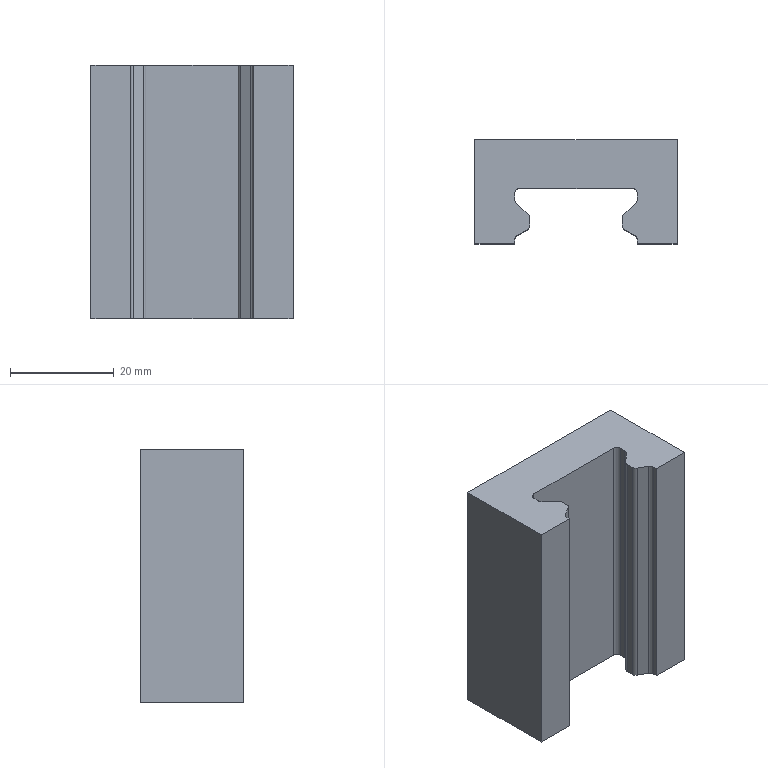Component | SolidWorks | MirrorSlider-2 | 1 solid | 28 faces | box 38.92 x 20 x 48.81 mm | volume 27036 mm3 | plane 18 | cylinder 10 | commonest cylinder face diameters 2 x10
STEP:
#1=COLOUR_RGB('',0.7922,0.8196,0.9333);
#2=FILL_AREA_STYLE_COLOUR('',#1);
#3=FILL_AREA_STYLE('',(#2));
#4=SURFACE_STYLE_FILL_AREA(#3);
#5=SURFACE_SIDE_STYLE('',(#4));
#6=SURFACE_STYLE_USAGE(.BOTH.,#5);
#7=PRESENTATION_STYLE_ASSIGNMENT((#6));
#8=CARTESIAN_POINT('',(-1.467,-8.441,-7.67));
#9=VERTEX_POINT('',#8);
#10=CARTESIAN_POINT('',(-1.467,-8.471,-7.67));
#11=VERTEX_POINT('',#10);
#12=CARTESIAN_POINT('',(-1.467,-7.683,-7.67));
#13=DIRECTION('',(0.,-1.,0.));
#14=VECTOR('',#13,39.37);
#15=LINE('',#12,#14);
#16=EDGE_CURVE('',#9,#11,#15,.T.);
#17=ORIENTED_EDGE('',*,*,#16,.F.);
#18=CARTESIAN_POINT('',(-1.486,-8.407,-7.67));
#19=VERTEX_POINT('',#18);
#20=CARTESIAN_POINT('',(-1.506,-8.441,-7.67));
#21=DIRECTION('',(0.,0.,1.));
#22=DIRECTION('',(0.,1.,0.));
#23=AXIS2_PLACEMENT_3D('',#20,#21,#22);
#24=CIRCLE('',#23,0.03937);
#25=EDGE_CURVE('',#9,#19,#24,.T.);
#26=ORIENTED_EDGE('',*,*,#25,.T.);
#27=CARTESIAN_POINT('',(-1.562,-8.363,-7.67));
#28=VERTEX_POINT('',#27);
#29=CARTESIAN_POINT('',(-0.6816,-8.869,-7.67));
#30=DIRECTION('',(0.8671,-0.4982,0.));
#31=VECTOR('',#30,39.37);
#32=LINE('',#29,#31);
#33=EDGE_CURVE('',#28,#19,#32,.T.);
#34=ORIENTED_EDGE('',*,*,#33,.F.);
#35=CARTESIAN_POINT('',(-1.582,-8.329,-7.67));
#36=VERTEX_POINT('',#35);
#37=CARTESIAN_POINT('',(-1.543,-8.329,-7.67));
#38=DIRECTION('',(0.,0.,1.));
#39=DIRECTION('',(0.,1.,0.));
#40=AXIS2_PLACEMENT_3D('',#37,#38,#39);
#41=CIRCLE('',#40,0.03937);
#42=EDGE_CURVE('',#36,#28,#41,.T.);
#43=ORIENTED_EDGE('',*,*,#42,.F.);
#44=CARTESIAN_POINT('',(-1.582,-8.278,-7.67));
#45=VERTEX_POINT('',#44);
#46=CARTESIAN_POINT('',(-1.582,-7.683,-7.67));
#47=DIRECTION('',(0.,-1.,0.));
#48=VECTOR('',#47,39.37);
#49=LINE('',#46,#48);
#50=EDGE_CURVE('',#45,#36,#49,.T.);
#51=ORIENTED_EDGE('',*,*,#50,.F.);
#52=CARTESIAN_POINT('',(-1.57,-8.249,-7.67));
#53=VERTEX_POINT('',#52);
#54=CARTESIAN_POINT('',(-1.543,-8.278,-7.67));
#55=DIRECTION('',(0.,0.,-1.));
#56=DIRECTION('',(0.,1.,0.));
#57=AXIS2_PLACEMENT_3D('',#54,#55,#56);
#58=CIRCLE('',#57,0.03937);
#59=EDGE_CURVE('',#45,#53,#58,.T.);
#60=ORIENTED_EDGE('',*,*,#59,.T.);
#61=CARTESIAN_POINT('',(-1.479,-8.164,-7.67));
#62=VERTEX_POINT('',#61);
#63=CARTESIAN_POINT('',(-0.4484,-7.203,-7.67));
#64=DIRECTION('',(-0.7311,-0.6823,0.));
#65=VECTOR('',#64,39.37);
#66=LINE('',#63,#65);
#67=EDGE_CURVE('',#62,#53,#66,.T.);
#68=ORIENTED_EDGE('',*,*,#67,.F.);
#69=CARTESIAN_POINT('',(-1.467,-8.136,-7.67));
#70=VERTEX_POINT('',#69);
#71=CARTESIAN_POINT('',(-1.506,-8.136,-7.67));
#72=DIRECTION('',(0.,0.,1.));
#73=DIRECTION('',(0.,1.,0.));
#74=AXIS2_PLACEMENT_3D('',#71,#72,#73);
#75=CIRCLE('',#74,0.03937);
#76=EDGE_CURVE('',#62,#70,#75,.T.);
#77=ORIENTED_EDGE('',*,*,#76,.T.);
#78=CARTESIAN_POINT('',(-1.467,-8.09,-7.67));
#79=VERTEX_POINT('',#78);
#80=CARTESIAN_POINT('',(-1.467,-7.683,-7.67));
#81=DIRECTION('',(0.,-1.,0.));
#82=VECTOR('',#81,39.37);
#83=LINE('',#80,#82);
#84=EDGE_CURVE('',#79,#70,#83,.T.);
#85=ORIENTED_EDGE('',*,*,#84,.F.);
#86=CARTESIAN_POINT('',(-1.506,-8.051,-7.67));
#87=VERTEX_POINT('',#86);
#88=CARTESIAN_POINT('',(-1.506,-8.09,-7.67));
#89=DIRECTION('',(0.,0.,-1.));
#90=DIRECTION('',(0.,1.,0.));
#91=AXIS2_PLACEMENT_3D('',#88,#89,#90);
#92=CIRCLE('',#91,0.03937);
#93=EDGE_CURVE('',#87,#79,#92,.T.);
#94=ORIENTED_EDGE('',*,*,#93,.F.);
#95=CARTESIAN_POINT('',(-2.356,-8.051,-7.67));
#96=VERTEX_POINT('',#95);
#97=CARTESIAN_POINT('',(-0.,-8.051,-7.67));
#98=DIRECTION('',(-1.,0.,0.));
#99=VECTOR('',#98,39.37);
#100=LINE('',#97,#99);
#101=EDGE_CURVE('',#87,#96,#100,.T.);
#102=ORIENTED_EDGE('',*,*,#101,.T.);
#103=CARTESIAN_POINT('',(-2.396,-8.09,-7.67));
#104=VERTEX_POINT('',#103);
#105=CARTESIAN_POINT('',(-2.356,-8.09,-7.67));
#106=DIRECTION('',(0.,0.,1.));
#107=DIRECTION('',(0.,1.,0.));
#108=AXIS2_PLACEMENT_3D('',#105,#106,#107);
#109=CIRCLE('',#108,0.03937);
#110=EDGE_CURVE('',#96,#104,#109,.T.);
#111=ORIENTED_EDGE('',*,*,#110,.T.);
#112=CARTESIAN_POINT('',(-2.396,-8.136,-7.67));
#113=VERTEX_POINT('',#112);
#114=CARTESIAN_POINT('',(-2.396,-7.683,-7.67));
#115=DIRECTION('',(0.,-1.,0.));
#116=VECTOR('',#115,39.37);
#117=LINE('',#114,#116);
#118=EDGE_CURVE('',#104,#113,#117,.T.);
#119=ORIENTED_EDGE('',*,*,#118,.T.);
#120=CARTESIAN_POINT('',(-2.383,-8.164,-7.67));
#121=VERTEX_POINT('',#120);
#122=CARTESIAN_POINT('',(-2.356,-8.136,-7.67));
#123=DIRECTION('',(0.,0.,-1.));
#124=DIRECTION('',(0.,1.,0.));
#125=AXIS2_PLACEMENT_3D('',#122,#123,#124);
#126=CIRCLE('',#125,0.03937);
#127=EDGE_CURVE('',#121,#113,#126,.T.);
#128=ORIENTED_EDGE('',*,*,#127,.F.);
#129=CARTESIAN_POINT('',(-2.292,-8.249,-7.67));
#130=VERTEX_POINT('',#129);
#131=CARTESIAN_POINT('',(-1.349,-9.129,-7.67));
#132=DIRECTION('',(0.7311,-0.6823,0.));
#133=VECTOR('',#132,39.37);
#134=LINE('',#131,#133);
#135=EDGE_CURVE('',#121,#130,#134,.T.);
#136=ORIENTED_EDGE('',*,*,#135,.T.);
#137=CARTESIAN_POINT('',(-2.28,-8.278,-7.67));
#138=VERTEX_POINT('',#137);
#139=CARTESIAN_POINT('',(-2.319,-8.278,-7.67));
#140=DIRECTION('',(0.,0.,1.));
#141=DIRECTION('',(0.,1.,0.));
#142=AXIS2_PLACEMENT_3D('',#139,#140,#141);
#143=CIRCLE('',#142,0.03937);
#144=EDGE_CURVE('',#138,#130,#143,.T.);
#145=ORIENTED_EDGE('',*,*,#144,.F.);
#146=CARTESIAN_POINT('',(-2.28,-8.329,-7.67));
#147=VERTEX_POINT('',#146);
#148=CARTESIAN_POINT('',(-2.28,-7.683,-7.67));
#149=DIRECTION('',(0.,-1.,0.));
#150=VECTOR('',#149,39.37);
#151=LINE('',#148,#150);
#152=EDGE_CURVE('',#138,#147,#151,.T.);
#153=ORIENTED_EDGE('',*,*,#152,.T.);
#154=CARTESIAN_POINT('',(-2.3,-8.363,-7.67));
#155=VERTEX_POINT('',#154);
#156=CARTESIAN_POINT('',(-2.319,-8.329,-7.67));
#157=DIRECTION('',(0.,0.,-1.));
#158=DIRECTION('',(0.,1.,0.));
#159=AXIS2_PLACEMENT_3D('',#156,#157,#158);
#160=CIRCLE('',#159,0.03937);
#161=EDGE_CURVE('',#147,#155,#160,.T.);
#162=ORIENTED_EDGE('',*,*,#161,.T.);
#163=CARTESIAN_POINT('',(-2.376,-8.407,-7.67));
#164=VERTEX_POINT('',#163);
#165=CARTESIAN_POINT('',(-0.2769,-7.201,-7.67));
#166=DIRECTION('',(-0.8671,-0.4982,0.));
#167=VECTOR('',#166,39.37);
#168=LINE('',#165,#167);
#169=EDGE_CURVE('',#155,#164,#168,.T.);
#170=ORIENTED_EDGE('',*,*,#169,.T.);
#171=CARTESIAN_POINT('',(-2.396,-8.441,-7.67));
#172=VERTEX_POINT('',#171);
#173=CARTESIAN_POINT('',(-2.356,-8.441,-7.67));
#174=DIRECTION('',(0.,0.,-1.));
#175=DIRECTION('',(0.,1.,0.));
#176=AXIS2_PLACEMENT_3D('',#173,#174,#175);
#177=CIRCLE('',#176,0.03937);
#178=EDGE_CURVE('',#172,#164,#177,.T.);
#179=ORIENTED_EDGE('',*,*,#178,.F.);
#180=CARTESIAN_POINT('',(-2.396,-8.471,-7.67));
#181=VERTEX_POINT('',#180);
#182=CARTESIAN_POINT('',(-2.396,-7.683,-7.67));
#183=DIRECTION('',(0.,-1.,0.));
#184=VECTOR('',#183,39.37);
#185=LINE('',#182,#184);
#186=EDGE_CURVE('',#172,#181,#185,.T.);
#187=ORIENTED_EDGE('',*,*,#186,.T.);
#188=CARTESIAN_POINT('',(-2.697,-8.471,-7.67));
#189=VERTEX_POINT('',#188);
#190=CARTESIAN_POINT('',(-1.165,-8.471,-7.67));
#191=DIRECTION('',(-1.,0.,0.));
#192=VECTOR('',#191,39.37);
#193=LINE('',#190,#192);
#194=EDGE_CURVE('',#181,#189,#193,.T.);
#195=ORIENTED_EDGE('',*,*,#194,.T.);
#196=CARTESIAN_POINT('',(-2.697,-7.683,-7.67));
#197=VERTEX_POINT('',#196);
#198=CARTESIAN_POINT('',(-2.697,-8.471,-7.67));
#199=DIRECTION('',(0.,1.,0.));
#200=VECTOR('',#199,39.37);
#201=LINE('',#198,#200);
#202=EDGE_CURVE('',#189,#197,#201,.T.);
#203=ORIENTED_EDGE('',*,*,#202,.T.);
#204=CARTESIAN_POINT('',(-1.165,-7.683,-7.67));
#205=VERTEX_POINT('',#204);
#206=CARTESIAN_POINT('',(-1.165,-7.683,-7.67));
#207=DIRECTION('',(-1.,0.,0.));
#208=VECTOR('',#207,39.37);
#209=LINE('',#206,#208);
#210=EDGE_CURVE('',#205,#197,#209,.T.);
#211=ORIENTED_EDGE('',*,*,#210,.F.);
#212=CARTESIAN_POINT('',(-1.165,-8.471,-7.67));
#213=VERTEX_POINT('',#212);
#214=CARTESIAN_POINT('',(-1.165,-8.471,-7.67));
#215=DIRECTION('',(0.,1.,0.));
#216=VECTOR('',#215,39.37);
#217=LINE('',#214,#216);
#218=EDGE_CURVE('',#213,#205,#217,.T.);
#219=ORIENTED_EDGE('',*,*,#218,.F.);
#220=CARTESIAN_POINT('',(-1.165,-8.471,-7.67));
#221=DIRECTION('',(-1.,0.,0.));
#222=VECTOR('',#221,39.37);
#223=LINE('',#220,#222);
#224=EDGE_CURVE('',#213,#11,#223,.T.);
#225=ORIENTED_EDGE('',*,*,#224,.T.);
#226=EDGE_LOOP('',(#17,#26,#34,#43,#51,#60,#68,#77,#85,#94,#102,#111,#119,#128,#136,#145,#153,#162,#170,#179,#187,#195,#203,#211,#219,#225));
#227=FACE_OUTER_BOUND('',#226,.T.);
#228=CARTESIAN_POINT('',(-1.165,-8.471,-7.67));
#229=DIRECTION('',(0.,0.,1.));
#230=DIRECTION('',(0.,-1.,0.));
#231=AXIS2_PLACEMENT_3D('',#228,#229,#230);
#232=PLANE('',#231);
#233=ADVANCED_FACE('',(#227),#232,.F.);
#234=CARTESIAN_POINT('',(-1.467,-8.441,-5.748));
#235=VERTEX_POINT('',#234);
#236=CARTESIAN_POINT('',(-1.467,-8.471,-5.748));
#237=VERTEX_POINT('',#236);
#238=CARTESIAN_POINT('',(-1.467,-8.471,-5.748));
#239=DIRECTION('',(0.,-1.,0.));
#240=VECTOR('',#239,39.37);
#241=LINE('',#238,#240);
#242=EDGE_CURVE('',#235,#237,#241,.T.);
#243=ORIENTED_EDGE('',*,*,#242,.T.);
#244=CARTESIAN_POINT('',(-1.165,-8.471,-5.748));
#245=VERTEX_POINT('',#244);
#246=CARTESIAN_POINT('',(-2.697,-8.471,-5.748));
#247=DIRECTION('',(1.,-0.,0.));
#248=VECTOR('',#247,39.37);
#249=LINE('',#246,#248);
#250=EDGE_CURVE('',#237,#245,#249,.T.);
#251=ORIENTED_EDGE('',*,*,#250,.T.);
#252=CARTESIAN_POINT('',(-1.165,-7.683,-5.748));
#253=VERTEX_POINT('',#252);
#254=CARTESIAN_POINT('',(-1.165,-8.471,-5.748));
#255=DIRECTION('',(0.,1.,0.));
#256=VECTOR('',#255,39.37);
#257=LINE('',#254,#256);
#258=EDGE_CURVE('',#245,#253,#257,.T.);
#259=ORIENTED_EDGE('',*,*,#258,.T.);
#260=CARTESIAN_POINT('',(-2.697,-7.683,-5.748));
#261=VERTEX_POINT('',#260);
#262=CARTESIAN_POINT('',(-2.697,-7.683,-5.748));
#263=DIRECTION('',(1.,-0.,0.));
#264=VECTOR('',#263,39.37);
#265=LINE('',#262,#264);
#266=EDGE_CURVE('',#261,#253,#265,.T.);
#267=ORIENTED_EDGE('',*,*,#266,.F.);
#268=CARTESIAN_POINT('',(-2.697,-8.471,-5.748));
#269=VERTEX_POINT('',#268);
#270=CARTESIAN_POINT('',(-2.697,-8.471,-5.748));
#271=DIRECTION('',(0.,1.,0.));
#272=VECTOR('',#271,39.37);
#273=LINE('',#270,#272);
#274=EDGE_CURVE('',#269,#261,#273,.T.);
#275=ORIENTED_EDGE('',*,*,#274,.F.);
#276=CARTESIAN_POINT('',(-2.396,-8.471,-5.748));
#277=VERTEX_POINT('',#276);
#278=CARTESIAN_POINT('',(-2.697,-8.471,-5.748));
#279=DIRECTION('',(1.,-0.,0.));
#280=VECTOR('',#279,39.37);
#281=LINE('',#278,#280);
#282=EDGE_CURVE('',#269,#277,#281,.T.);
#283=ORIENTED_EDGE('',*,*,#282,.T.);
#284=CARTESIAN_POINT('',(-2.396,-8.441,-5.748));
#285=VERTEX_POINT('',#284);
#286=CARTESIAN_POINT('',(-2.396,-8.471,-5.748));
#287=DIRECTION('',(0.,-1.,0.));
#288=VECTOR('',#287,39.37);
#289=LINE('',#286,#288);
#290=EDGE_CURVE('',#285,#277,#289,.T.);
#291=ORIENTED_EDGE('',*,*,#290,.F.);
#292=CARTESIAN_POINT('',(-2.376,-8.407,-5.748));
#293=VERTEX_POINT('',#292);
#294=CARTESIAN_POINT('',(-2.356,-8.441,-5.748));
#295=DIRECTION('',(0.,0.,-1.));
#296=DIRECTION('',(0.,1.,0.));
#297=AXIS2_PLACEMENT_3D('',#294,#295,#296);
#298=CIRCLE('',#297,0.03937);
#299=EDGE_CURVE('',#285,#293,#298,.T.);
#300=ORIENTED_EDGE('',*,*,#299,.T.);
#301=CARTESIAN_POINT('',(-2.3,-8.363,-5.748));
#302=VERTEX_POINT('',#301);
#303=CARTESIAN_POINT('',(-2.645,-8.562,-5.748));
#304=DIRECTION('',(-0.8671,-0.4982,0.));
#305=VECTOR('',#304,39.37);
#306=LINE('',#303,#305);
#307=EDGE_CURVE('',#302,#293,#306,.T.);
#308=ORIENTED_EDGE('',*,*,#307,.F.);
#309=CARTESIAN_POINT('',(-2.28,-8.329,-5.748));
#310=VERTEX_POINT('',#309);
#311=CARTESIAN_POINT('',(-2.319,-8.329,-5.748));
#312=DIRECTION('',(0.,0.,-1.));
#313=DIRECTION('',(0.,1.,0.));
#314=AXIS2_PLACEMENT_3D('',#311,#312,#313);
#315=CIRCLE('',#314,0.03937);
#316=EDGE_CURVE('',#310,#302,#315,.T.);
#317=ORIENTED_EDGE('',*,*,#316,.F.);
#318=CARTESIAN_POINT('',(-2.28,-8.278,-5.748));
#319=VERTEX_POINT('',#318);
#320=CARTESIAN_POINT('',(-2.28,-8.471,-5.748));
#321=DIRECTION('',(0.,-1.,0.));
#322=VECTOR('',#321,39.37);
#323=LINE('',#320,#322);
#324=EDGE_CURVE('',#319,#310,#323,.T.);
#325=ORIENTED_EDGE('',*,*,#324,.F.);
#326=CARTESIAN_POINT('',(-2.292,-8.249,-5.748));
#327=VERTEX_POINT('',#326);
#328=CARTESIAN_POINT('',(-2.319,-8.278,-5.748));
#329=DIRECTION('',(0.,0.,1.));
#330=DIRECTION('',(0.,1.,0.));
#331=AXIS2_PLACEMENT_3D('',#328,#329,#330);
#332=CIRCLE('',#331,0.03937);
#333=EDGE_CURVE('',#319,#327,#332,.T.);
#334=ORIENTED_EDGE('',*,*,#333,.T.);
#335=CARTESIAN_POINT('',(-2.383,-8.164,-5.748));
#336=VERTEX_POINT('',#335);
#337=CARTESIAN_POINT('',(-2.398,-8.15,-5.748));
#338=DIRECTION('',(0.7311,-0.6823,0.));
#339=VECTOR('',#338,39.37);
#340=LINE('',#337,#339);
#341=EDGE_CURVE('',#336,#327,#340,.T.);
#342=ORIENTED_EDGE('',*,*,#341,.F.);
#343=CARTESIAN_POINT('',(-2.396,-8.136,-5.748));
#344=VERTEX_POINT('',#343);
#345=CARTESIAN_POINT('',(-2.356,-8.136,-5.748));
#346=DIRECTION('',(0.,0.,-1.));
#347=DIRECTION('',(0.,1.,0.));
#348=AXIS2_PLACEMENT_3D('',#345,#346,#347);
#349=CIRCLE('',#348,0.03937);
#350=EDGE_CURVE('',#336,#344,#349,.T.);
#351=ORIENTED_EDGE('',*,*,#350,.T.);
#352=CARTESIAN_POINT('',(-2.396,-8.09,-5.748));
#353=VERTEX_POINT('',#352);
#354=CARTESIAN_POINT('',(-2.396,-8.471,-5.748));
#355=DIRECTION('',(0.,-1.,0.));
#356=VECTOR('',#355,39.37);
#357=LINE('',#354,#356);
#358=EDGE_CURVE('',#353,#344,#357,.T.);
#359=ORIENTED_EDGE('',*,*,#358,.F.);
#360=CARTESIAN_POINT('',(-2.356,-8.051,-5.748));
#361=VERTEX_POINT('',#360);
#362=CARTESIAN_POINT('',(-2.356,-8.09,-5.748));
#363=DIRECTION('',(0.,0.,1.));
#364=DIRECTION('',(0.,1.,0.));
#365=AXIS2_PLACEMENT_3D('',#362,#363,#364);
#366=CIRCLE('',#365,0.03937);
#367=EDGE_CURVE('',#361,#353,#366,.T.);
#368=ORIENTED_EDGE('',*,*,#367,.F.);
#369=CARTESIAN_POINT('',(-1.506,-8.051,-5.748));
#370=VERTEX_POINT('',#369);
#371=CARTESIAN_POINT('',(-2.697,-8.051,-5.748));
#372=DIRECTION('',(-1.,0.,0.));
#373=VECTOR('',#372,39.37);
#374=LINE('',#371,#373);
#375=EDGE_CURVE('',#370,#361,#374,.T.);
#376=ORIENTED_EDGE('',*,*,#375,.F.);
#377=CARTESIAN_POINT('',(-1.467,-8.09,-5.748));
#378=VERTEX_POINT('',#377);
#379=CARTESIAN_POINT('',(-1.506,-8.09,-5.748));
#380=DIRECTION('',(0.,0.,-1.));
#381=DIRECTION('',(0.,1.,0.));
#382=AXIS2_PLACEMENT_3D('',#379,#380,#381);
#383=CIRCLE('',#382,0.03937);
#384=EDGE_CURVE('',#370,#378,#383,.T.);
#385=ORIENTED_EDGE('',*,*,#384,.T.);
#386=CARTESIAN_POINT('',(-1.467,-8.136,-5.748));
#387=VERTEX_POINT('',#386);
#388=CARTESIAN_POINT('',(-1.467,-8.471,-5.748));
#389=DIRECTION('',(0.,-1.,0.));
#390=VECTOR('',#389,39.37);
#391=LINE('',#388,#390);
#392=EDGE_CURVE('',#378,#387,#391,.T.);
#393=ORIENTED_EDGE('',*,*,#392,.T.);
#394=CARTESIAN_POINT('',(-1.479,-8.164,-5.748));
#395=VERTEX_POINT('',#394);
#396=CARTESIAN_POINT('',(-1.506,-8.136,-5.748));
#397=DIRECTION('',(0.,0.,1.));
#398=DIRECTION('',(0.,1.,0.));
#399=AXIS2_PLACEMENT_3D('',#396,#397,#398);
#400=CIRCLE('',#399,0.03937);
#401=EDGE_CURVE('',#395,#387,#400,.T.);
#402=ORIENTED_EDGE('',*,*,#401,.F.);
#403=CARTESIAN_POINT('',(-1.57,-8.249,-5.748));
#404=VERTEX_POINT('',#403);
#405=CARTESIAN_POINT('',(-2.283,-8.915,-5.748));
#406=DIRECTION('',(-0.7311,-0.6823,0.));
#407=VECTOR('',#406,39.37);
#408=LINE('',#405,#407);
#409=EDGE_CURVE('',#395,#404,#408,.T.);
#410=ORIENTED_EDGE('',*,*,#409,.T.);
#411=CARTESIAN_POINT('',(-1.582,-8.278,-5.748));
#412=VERTEX_POINT('',#411);
#413=CARTESIAN_POINT('',(-1.543,-8.278,-5.748));
#414=DIRECTION('',(0.,0.,-1.));
#415=DIRECTION('',(0.,1.,0.));
#416=AXIS2_PLACEMENT_3D('',#413,#414,#415);
#417=CIRCLE('',#416,0.03937);
#418=EDGE_CURVE('',#412,#404,#417,.T.);
#419=ORIENTED_EDGE('',*,*,#418,.F.);
#420=CARTESIAN_POINT('',(-1.582,-8.329,-5.748));
#421=VERTEX_POINT('',#420);
#422=CARTESIAN_POINT('',(-1.582,-8.471,-5.748));
#423=DIRECTION('',(0.,-1.,0.));
#424=VECTOR('',#423,39.37);
#425=LINE('',#422,#424);
#426=EDGE_CURVE('',#412,#421,#425,.T.);
#427=ORIENTED_EDGE('',*,*,#426,.T.);
#428=CARTESIAN_POINT('',(-1.562,-8.363,-5.748));
#429=VERTEX_POINT('',#428);
#430=CARTESIAN_POINT('',(-1.543,-8.329,-5.748));
#431=DIRECTION('',(0.,0.,1.));
#432=DIRECTION('',(0.,1.,0.));
#433=AXIS2_PLACEMENT_3D('',#430,#431,#432);
#434=CIRCLE('',#433,0.03937);
#435=EDGE_CURVE('',#421,#429,#434,.T.);
#436=ORIENTED_EDGE('',*,*,#435,.T.);
#437=CARTESIAN_POINT('',(-1.486,-8.407,-5.748));
#438=VERTEX_POINT('',#437);
#439=CARTESIAN_POINT('',(-2.369,-7.9,-5.748));
#440=DIRECTION('',(0.8671,-0.4982,0.));
#441=VECTOR('',#440,39.37);
#442=LINE('',#439,#441);
#443=EDGE_CURVE('',#429,#438,#442,.T.);
#444=ORIENTED_EDGE('',*,*,#443,.T.);
#445=CARTESIAN_POINT('',(-1.506,-8.441,-5.748));
#446=DIRECTION('',(0.,0.,1.));
#447=DIRECTION('',(0.,1.,0.));
#448=AXIS2_PLACEMENT_3D('',#445,#446,#447);
#449=CIRCLE('',#448,0.03937);
#450=EDGE_CURVE('',#235,#438,#449,.T.);
#451=ORIENTED_EDGE('',*,*,#450,.F.);
#452=EDGE_LOOP('',(#243,#251,#259,#267,#275,#283,#291,#300,#308,#317,#325,#334,#342,#351,#359,#368,#376,#385,#393,#402,#410,#419,#427,#436,#444,#451));
#453=FACE_OUTER_BOUND('',#452,.T.);
#454=CARTESIAN_POINT('',(-2.697,-8.471,-5.748));
#455=DIRECTION('',(0.,0.,-1.));
#456=DIRECTION('',(0.,1.,0.));
#457=AXIS2_PLACEMENT_3D('',#454,#455,#456);
#458=PLANE('',#457);
#459=ADVANCED_FACE('',(#453),#458,.F.);
#460=ORIENTED_EDGE('',*,*,#224,.F.);
#461=CARTESIAN_POINT('',(-1.165,-8.471,-5.748));
#462=DIRECTION('',(-0.,0.,-1.));
#463=VECTOR('',#462,39.37);
#464=LINE('',#461,#463);
#465=EDGE_CURVE('',#245,#213,#464,.T.);
#466=ORIENTED_EDGE('',*,*,#465,.F.);
#467=ORIENTED_EDGE('',*,*,#250,.F.);
#468=CARTESIAN_POINT('',(-1.467,-8.471,-5.748));
#469=DIRECTION('',(0.,0.,1.));
#470=VECTOR('',#469,39.37);
#471=LINE('',#468,#470);
#472=EDGE_CURVE('',#11,#237,#471,.T.);
#473=ORIENTED_EDGE('',*,*,#472,.F.);
#474=EDGE_LOOP('',(#460,#466,#467,#473));
#475=FACE_OUTER_BOUND('',#474,.T.);
#476=CARTESIAN_POINT('',(-0.,-8.471,-5.748));
#477=DIRECTION('',(-0.,-1.,0.));
#478=DIRECTION('',(-1.,0.,0.));
#479=AXIS2_PLACEMENT_3D('',#476,#477,#478);
#480=PLANE('',#479);
#481=ADVANCED_FACE('',(#475),#480,.T.);
#482=CARTESIAN_POINT('',(-2.697,-7.683,-7.67));
#483=DIRECTION('',(0.,0.,1.));
#484=VECTOR('',#483,39.37);
#485=LINE('',#482,#484);
#486=EDGE_CURVE('',#197,#261,#485,.T.);
#487=ORIENTED_EDGE('',*,*,#486,.F.);
#488=ORIENTED_EDGE('',*,*,#202,.F.);
#489=CARTESIAN_POINT('',(-2.697,-8.471,-7.67));
#490=DIRECTION('',(0.,0.,1.));
#491=VECTOR('',#490,39.37);
#492=LINE('',#489,#491);
#493=EDGE_CURVE('',#189,#269,#492,.T.);
#494=ORIENTED_EDGE('',*,*,#493,.T.);
#495=ORIENTED_EDGE('',*,*,#274,.T.);
#496=EDGE_LOOP('',(#487,#488,#494,#495));
#497=FACE_OUTER_BOUND('',#496,.T.);
#498=CARTESIAN_POINT('',(-2.697,-8.471,-7.67));
#499=DIRECTION('',(1.,0.,0.));
#500=DIRECTION('',(0.,-1.,0.));
#501=AXIS2_PLACEMENT_3D('',#498,#499,#500);
#502=PLANE('',#501);
#503=ADVANCED_FACE('',(#497),#502,.F.);
#504=CARTESIAN_POINT('',(-1.165,-7.683,-5.748));
#505=DIRECTION('',(-0.,0.,-1.));
#506=VECTOR('',#505,39.37);
#507=LINE('',#504,#506);
#508=EDGE_CURVE('',#253,#205,#507,.T.);
#509=ORIENTED_EDGE('',*,*,#508,.F.);
#510=ORIENTED_EDGE('',*,*,#258,.F.);
#511=ORIENTED_EDGE('',*,*,#465,.T.);
#512=ORIENTED_EDGE('',*,*,#218,.T.);
#513=EDGE_LOOP('',(#509,#510,#511,#512));
#514=FACE_OUTER_BOUND('',#513,.T.);
#515=CARTESIAN_POINT('',(-1.165,-8.471,-5.748));
#516=DIRECTION('',(-1.,0.,0.));
#517=DIRECTION('',(0.,-0.,1.));
#518=AXIS2_PLACEMENT_3D('',#515,#516,#517);
#519=PLANE('',#518);
#520=ADVANCED_FACE('',(#514),#519,.F.);
#521=CARTESIAN_POINT('',(-2.396,-8.471,-5.748));
#522=DIRECTION('',(0.,0.,1.));
#523=VECTOR('',#522,39.37);
#524=LINE('',#521,#523);
#525=EDGE_CURVE('',#181,#277,#524,.T.);
#526=ORIENTED_EDGE('',*,*,#525,.T.);
#527=ORIENTED_EDGE('',*,*,#282,.F.);
#528=ORIENTED_EDGE('',*,*,#493,.F.);
#529=ORIENTED_EDGE('',*,*,#194,.F.);
#530=EDGE_LOOP('',(#526,#527,#528,#529));
#531=FACE_OUTER_BOUND('',#530,.T.);
#532=CARTESIAN_POINT('',(-0.,-8.471,-5.748));
#533=DIRECTION('',(-0.,-1.,0.));
#534=DIRECTION('',(-1.,0.,0.));
#535=AXIS2_PLACEMENT_3D('',#532,#533,#534);
#536=PLANE('',#535);
#537=ADVANCED_FACE('',(#531),#536,.T.);
#538=ORIENTED_EDGE('',*,*,#210,.T.);
#539=ORIENTED_EDGE('',*,*,#486,.T.);
#540=ORIENTED_EDGE('',*,*,#266,.T.);
#541=ORIENTED_EDGE('',*,*,#508,.T.);
#542=EDGE_LOOP('',(#538,#539,#540,#541));
#543=FACE_OUTER_BOUND('',#542,.T.);
#544=CARTESIAN_POINT('',(-0.,-7.683,-5.748));
#545=DIRECTION('',(-0.,-1.,0.));
#546=DIRECTION('',(-1.,0.,0.));
#547=AXIS2_PLACEMENT_3D('',#544,#545,#546);
#548=PLANE('',#547);
#549=ADVANCED_FACE('',(#543),#548,.F.);
#550=ORIENTED_EDGE('',*,*,#350,.F.);
#551=CARTESIAN_POINT('',(-2.383,-8.164,-4.993));
#552=DIRECTION('',(0.,0.,-1.));
#553=VECTOR('',#552,39.37);
#554=LINE('',#551,#553);
#555=EDGE_CURVE('',#336,#121,#554,.T.);
#556=ORIENTED_EDGE('',*,*,#555,.T.);
#557=ORIENTED_EDGE('',*,*,#127,.T.);
#558=CARTESIAN_POINT('',(-2.396,-8.136,-4.993));
#559=DIRECTION('',(0.,0.,-1.));
#560=VECTOR('',#559,39.37);
#561=LINE('',#558,#560);
#562=EDGE_CURVE('',#344,#113,#561,.T.);
#563=ORIENTED_EDGE('',*,*,#562,.F.);
#564=EDGE_LOOP('',(#550,#556,#557,#563));
#565=FACE_OUTER_BOUND('',#564,.T.);
#566=CARTESIAN_POINT('',(-2.356,-8.136,-4.993));
#567=DIRECTION('',(0.,0.,-1.));
#568=DIRECTION('',(0.,1.,0.));
#569=AXIS2_PLACEMENT_3D('',#566,#567,#568);
#570=CYLINDRICAL_SURFACE('',#569,0.03937);
#571=ADVANCED_FACE('',(#565),#570,.F.);
#572=CARTESIAN_POINT('',(-2.396,-8.09,-4.993));
#573=DIRECTION('',(0.,0.,-1.));
#574=VECTOR('',#573,39.37);
#575=LINE('',#572,#574);
#576=EDGE_CURVE('',#353,#104,#575,.T.);
#577=ORIENTED_EDGE('',*,*,#576,.F.);
#578=ORIENTED_EDGE('',*,*,#358,.T.);
#579=ORIENTED_EDGE('',*,*,#562,.T.);
#580=ORIENTED_EDGE('',*,*,#118,.F.);
#581=EDGE_LOOP('',(#577,#578,#579,#580));
#582=FACE_OUTER_BOUND('',#581,.T.);
#583=CARTESIAN_POINT('',(-2.396,-7.683,-4.993));
#584=DIRECTION('',(-1.,0.,0.));
#585=DIRECTION('',(0.,1.,0.));
#586=AXIS2_PLACEMENT_3D('',#583,#584,#585);
#587=PLANE('',#586);
#588=ADVANCED_FACE('',(#582),#587,.F.);
#589=CARTESIAN_POINT('',(-2.356,-8.051,-4.993));
#590=DIRECTION('',(0.,0.,-1.));
#591=VECTOR('',#590,39.37);
#592=LINE('',#589,#591);
#593=EDGE_CURVE('',#361,#96,#592,.T.);
#594=ORIENTED_EDGE('',*,*,#593,.F.);
#595=ORIENTED_EDGE('',*,*,#367,.T.);
#596=ORIENTED_EDGE('',*,*,#576,.T.);
#597=ORIENTED_EDGE('',*,*,#110,.F.);
#598=EDGE_LOOP('',(#594,#595,#596,#597));
#599=FACE_OUTER_BOUND('',#598,.T.);
#600=CARTESIAN_POINT('',(-2.356,-8.09,-4.993));
#601=DIRECTION('',(0.,0.,-1.));
#602=DIRECTION('',(0.,1.,0.));
#603=AXIS2_PLACEMENT_3D('',#600,#601,#602);
#604=CYLINDRICAL_SURFACE('',#603,0.03937);
#605=ADVANCED_FACE('',(#599),#604,.F.);
#606=CARTESIAN_POINT('',(-1.506,-8.051,-4.993));
#607=DIRECTION('',(0.,0.,-1.));
#608=VECTOR('',#607,39.37);
#609=LINE('',#606,#608);
#610=EDGE_CURVE('',#370,#87,#609,.T.);
#611=ORIENTED_EDGE('',*,*,#610,.F.);
#612=ORIENTED_EDGE('',*,*,#375,.T.);
#613=ORIENTED_EDGE('',*,*,#593,.T.);
#614=ORIENTED_EDGE('',*,*,#101,.F.);
#615=EDGE_LOOP('',(#611,#612,#613,#614));
#616=FACE_OUTER_BOUND('',#615,.T.);
#617=CARTESIAN_POINT('',(-0.,-8.051,-4.993));
#618=DIRECTION('',(0.,1.,0.));
#619=DIRECTION('',(1.,-0.,0.));
#620=AXIS2_PLACEMENT_3D('',#617,#618,#619);
#621=PLANE('',#620);
#622=ADVANCED_FACE('',(#616),#621,.F.);
#623=ORIENTED_EDGE('',*,*,#384,.F.);
#624=ORIENTED_EDGE('',*,*,#610,.T.);
#625=ORIENTED_EDGE('',*,*,#93,.T.);
#626=CARTESIAN_POINT('',(-1.467,-8.09,-4.993));
#627=DIRECTION('',(0.,0.,-1.));
#628=VECTOR('',#627,39.37);
#629=LINE('',#626,#628);
#630=EDGE_CURVE('',#378,#79,#629,.T.);
#631=ORIENTED_EDGE('',*,*,#630,.F.);
#632=EDGE_LOOP('',(#623,#624,#625,#631));
#633=FACE_OUTER_BOUND('',#632,.T.);
#634=CARTESIAN_POINT('',(-1.506,-8.09,-4.993));
#635=DIRECTION('',(0.,0.,-1.));
#636=DIRECTION('',(0.,1.,0.));
#637=AXIS2_PLACEMENT_3D('',#634,#635,#636);
#638=CYLINDRICAL_SURFACE('',#637,0.03937);
#639=ADVANCED_FACE('',(#633),#638,.F.);
#640=ORIENTED_EDGE('',*,*,#392,.F.);
#641=ORIENTED_EDGE('',*,*,#630,.T.);
#642=ORIENTED_EDGE('',*,*,#84,.T.);
#643=CARTESIAN_POINT('',(-1.467,-8.136,-4.993));
#644=DIRECTION('',(0.,0.,-1.));
#645=VECTOR('',#644,39.37);
#646=LINE('',#643,#645);
#647=EDGE_CURVE('',#387,#70,#646,.T.);
#648=ORIENTED_EDGE('',*,*,#647,.F.);
#649=EDGE_LOOP('',(#640,#641,#642,#648));
#650=FACE_OUTER_BOUND('',#649,.T.);
#651=CARTESIAN_POINT('',(-1.467,-7.683,-4.993));
#652=DIRECTION('',(-1.,0.,0.));
#653=DIRECTION('',(0.,1.,0.));
#654=AXIS2_PLACEMENT_3D('',#651,#652,#653);
#655=PLANE('',#654);
#656=ADVANCED_FACE('',(#650),#655,.T.);
#657=CARTESIAN_POINT('',(-1.479,-8.164,-4.993));
#658=DIRECTION('',(0.,0.,-1.));
#659=VECTOR('',#658,39.37);
#660=LINE('',#657,#659);
#661=EDGE_CURVE('',#395,#62,#660,.T.);
#662=ORIENTED_EDGE('',*,*,#661,.F.);
#663=ORIENTED_EDGE('',*,*,#401,.T.);
#664=ORIENTED_EDGE('',*,*,#647,.T.);
#665=ORIENTED_EDGE('',*,*,#76,.F.);
#666=EDGE_LOOP('',(#662,#663,#664,#665));
#667=FACE_OUTER_BOUND('',#666,.T.);
#668=CARTESIAN_POINT('',(-1.506,-8.136,-4.993));
#669=DIRECTION('',(0.,0.,-1.));
#670=DIRECTION('',(0.,1.,0.));
#671=AXIS2_PLACEMENT_3D('',#668,#669,#670);
#672=CYLINDRICAL_SURFACE('',#671,0.03937);
#673=ADVANCED_FACE('',(#667),#672,.F.);
#674=ORIENTED_EDGE('',*,*,#409,.F.);
#675=ORIENTED_EDGE('',*,*,#661,.T.);
#676=ORIENTED_EDGE('',*,*,#67,.T.);
#677=CARTESIAN_POINT('',(-1.57,-8.249,-4.993));
#678=DIRECTION('',(0.,0.,-1.));
#679=VECTOR('',#678,39.37);
#680=LINE('',#677,#679);
#681=EDGE_CURVE('',#404,#53,#680,.T.);
#682=ORIENTED_EDGE('',*,*,#681,.F.);
#683=EDGE_LOOP('',(#674,#675,#676,#682));
#684=FACE_OUTER_BOUND('',#683,.T.);
#685=CARTESIAN_POINT('',(-0.4484,-7.203,-4.993));
#686=DIRECTION('',(-0.6823,0.7311,0.));
#687=DIRECTION('',(0.7311,0.6823,0.));
#688=AXIS2_PLACEMENT_3D('',#685,#686,#687);
#689=PLANE('',#688);
#690=ADVANCED_FACE('',(#684),#689,.T.);
#691=CARTESIAN_POINT('',(-1.582,-8.278,-4.993));
#692=DIRECTION('',(0.,0.,-1.));
#693=VECTOR('',#692,39.37);
#694=LINE('',#691,#693);
#695=EDGE_CURVE('',#412,#45,#694,.T.);
#696=ORIENTED_EDGE('',*,*,#695,.F.);
#697=ORIENTED_EDGE('',*,*,#418,.T.);
#698=ORIENTED_EDGE('',*,*,#681,.T.);
#699=ORIENTED_EDGE('',*,*,#59,.F.);
#700=EDGE_LOOP('',(#696,#697,#698,#699));
#701=FACE_OUTER_BOUND('',#700,.T.);
#702=CARTESIAN_POINT('',(-1.543,-8.278,-4.993));
#703=DIRECTION('',(0.,0.,-1.));
#704=DIRECTION('',(0.,1.,0.));
#705=AXIS2_PLACEMENT_3D('',#702,#703,#704);
#706=CYLINDRICAL_SURFACE('',#705,0.03937);
#707=ADVANCED_FACE('',(#701),#706,.T.);
#708=ORIENTED_EDGE('',*,*,#426,.F.);
#709=ORIENTED_EDGE('',*,*,#695,.T.);
#710=ORIENTED_EDGE('',*,*,#50,.T.);
#711=CARTESIAN_POINT('',(-1.582,-8.329,-4.993));
#712=DIRECTION('',(0.,0.,-1.));
#713=VECTOR('',#712,39.37);
#714=LINE('',#711,#713);
#715=EDGE_CURVE('',#421,#36,#714,.T.);
#716=ORIENTED_EDGE('',*,*,#715,.F.);
#717=EDGE_LOOP('',(#708,#709,#710,#716));
#718=FACE_OUTER_BOUND('',#717,.T.);
#719=CARTESIAN_POINT('',(-1.582,-7.683,-4.993));
#720=DIRECTION('',(-1.,0.,0.));
#721=DIRECTION('',(0.,1.,0.));
#722=AXIS2_PLACEMENT_3D('',#719,#720,#721);
#723=PLANE('',#722);
#724=ADVANCED_FACE('',(#718),#723,.T.);
#725=ORIENTED_EDGE('',*,*,#435,.F.);
#726=ORIENTED_EDGE('',*,*,#715,.T.);
#727=ORIENTED_EDGE('',*,*,#42,.T.);
#728=CARTESIAN_POINT('',(-1.562,-8.363,-4.993));
#729=DIRECTION('',(0.,0.,-1.));
#730=VECTOR('',#729,39.37);
#731=LINE('',#728,#730);
#732=EDGE_CURVE('',#429,#28,#731,.T.);
#733=ORIENTED_EDGE('',*,*,#732,.F.);
#734=EDGE_LOOP('',(#725,#726,#727,#733));
#735=FACE_OUTER_BOUND('',#734,.T.);
#736=CARTESIAN_POINT('',(-1.543,-8.329,-4.993));
#737=DIRECTION('',(0.,0.,-1.));
#738=DIRECTION('',(0.,1.,0.));
#739=AXIS2_PLACEMENT_3D('',#736,#737,#738);
#740=CYLINDRICAL_SURFACE('',#739,0.03937);
#741=ADVANCED_FACE('',(#735),#740,.T.);
#742=ORIENTED_EDGE('',*,*,#443,.F.);
#743=ORIENTED_EDGE('',*,*,#732,.T.);
#744=ORIENTED_EDGE('',*,*,#33,.T.);
#745=CARTESIAN_POINT('',(-1.486,-8.407,-4.993));
#746=DIRECTION('',(0.,0.,-1.));
#747=VECTOR('',#746,39.37);
#748=LINE('',#745,#747);
#749=EDGE_CURVE('',#438,#19,#748,.T.);
#750=ORIENTED_EDGE('',*,*,#749,.F.);
#751=EDGE_LOOP('',(#742,#743,#744,#750));
#752=FACE_OUTER_BOUND('',#751,.T.);
#753=CARTESIAN_POINT('',(-0.6816,-8.869,-4.993));
#754=DIRECTION('',(-0.4982,-0.8671,0.));
#755=DIRECTION('',(-0.8671,0.4982,0.));
#756=AXIS2_PLACEMENT_3D('',#753,#754,#755);
#757=PLANE('',#756);
#758=ADVANCED_FACE('',(#752),#757,.T.);
#759=CARTESIAN_POINT('',(-1.467,-8.441,-4.993));
#760=DIRECTION('',(0.,0.,-1.));
#761=VECTOR('',#760,39.37);
#762=LINE('',#759,#761);
#763=EDGE_CURVE('',#235,#9,#762,.T.);
#764=ORIENTED_EDGE('',*,*,#763,.F.);
#765=ORIENTED_EDGE('',*,*,#450,.T.);
#766=ORIENTED_EDGE('',*,*,#749,.T.);
#767=ORIENTED_EDGE('',*,*,#25,.F.);
#768=EDGE_LOOP('',(#764,#765,#766,#767));
#769=FACE_OUTER_BOUND('',#768,.T.);
#770=CARTESIAN_POINT('',(-1.506,-8.441,-4.993));
#771=DIRECTION('',(0.,0.,-1.));
#772=DIRECTION('',(0.,1.,0.));
#773=AXIS2_PLACEMENT_3D('',#770,#771,#772);
#774=CYLINDRICAL_SURFACE('',#773,0.03937);
#775=ADVANCED_FACE('',(#769),#774,.F.);
#776=ORIENTED_EDGE('',*,*,#299,.F.);
#777=CARTESIAN_POINT('',(-2.396,-8.441,-4.993));
#778=DIRECTION('',(0.,0.,-1.));
#779=VECTOR('',#778,39.37);
#780=LINE('',#777,#779);
#781=EDGE_CURVE('',#285,#172,#780,.T.);
#782=ORIENTED_EDGE('',*,*,#781,.T.);
#783=ORIENTED_EDGE('',*,*,#178,.T.);
#784=CARTESIAN_POINT('',(-2.376,-8.407,-4.993));
#785=DIRECTION('',(0.,0.,-1.));
#786=VECTOR('',#785,39.37);
#787=LINE('',#784,#786);
#788=EDGE_CURVE('',#293,#164,#787,.T.);
#789=ORIENTED_EDGE('',*,*,#788,.F.);
#790=EDGE_LOOP('',(#776,#782,#783,#789));
#791=FACE_OUTER_BOUND('',#790,.T.);
#792=CARTESIAN_POINT('',(-2.356,-8.441,-4.993));
#793=DIRECTION('',(0.,0.,-1.));
#794=DIRECTION('',(0.,1.,0.));
#795=AXIS2_PLACEMENT_3D('',#792,#793,#794);
#796=CYLINDRICAL_SURFACE('',#795,0.03937);
#797=ADVANCED_FACE('',(#791),#796,.F.);
#798=CARTESIAN_POINT('',(-2.3,-8.363,-4.993));
#799=DIRECTION('',(0.,0.,-1.));
#800=VECTOR('',#799,39.37);
#801=LINE('',#798,#800);
#802=EDGE_CURVE('',#302,#155,#801,.T.);
#803=ORIENTED_EDGE('',*,*,#802,.F.);
#804=ORIENTED_EDGE('',*,*,#307,.T.);
#805=ORIENTED_EDGE('',*,*,#788,.T.);
#806=ORIENTED_EDGE('',*,*,#169,.F.);
#807=EDGE_LOOP('',(#803,#804,#805,#806));
#808=FACE_OUTER_BOUND('',#807,.T.);
#809=CARTESIAN_POINT('',(-0.2769,-7.201,-4.993));
#810=DIRECTION('',(-0.4982,0.8671,0.));
#811=DIRECTION('',(0.8671,0.4982,0.));
#812=AXIS2_PLACEMENT_3D('',#809,#810,#811);
#813=PLANE('',#812);
#814=ADVANCED_FACE('',(#808),#813,.F.);
#815=CARTESIAN_POINT('',(-2.28,-8.329,-4.993));
#816=DIRECTION('',(0.,0.,-1.));
#817=VECTOR('',#816,39.37);
#818=LINE('',#815,#817);
#819=EDGE_CURVE('',#310,#147,#818,.T.);
#820=ORIENTED_EDGE('',*,*,#819,.F.);
#821=ORIENTED_EDGE('',*,*,#316,.T.);
#822=ORIENTED_EDGE('',*,*,#802,.T.);
#823=ORIENTED_EDGE('',*,*,#161,.F.);
#824=EDGE_LOOP('',(#820,#821,#822,#823));
#825=FACE_OUTER_BOUND('',#824,.T.);
#826=CARTESIAN_POINT('',(-2.319,-8.329,-4.993));
#827=DIRECTION('',(0.,0.,-1.));
#828=DIRECTION('',(0.,1.,0.));
#829=AXIS2_PLACEMENT_3D('',#826,#827,#828);
#830=CYLINDRICAL_SURFACE('',#829,0.03937);
#831=ADVANCED_FACE('',(#825),#830,.T.);
#832=CARTESIAN_POINT('',(-2.28,-8.278,-4.993));
#833=DIRECTION('',(0.,0.,-1.));
#834=VECTOR('',#833,39.37);
#835=LINE('',#832,#834);
#836=EDGE_CURVE('',#319,#138,#835,.T.);
#837=ORIENTED_EDGE('',*,*,#836,.F.);
#838=ORIENTED_EDGE('',*,*,#324,.T.);
#839=ORIENTED_EDGE('',*,*,#819,.T.);
#840=ORIENTED_EDGE('',*,*,#152,.F.);
#841=EDGE_LOOP('',(#837,#838,#839,#840));
#842=FACE_OUTER_BOUND('',#841,.T.);
#843=CARTESIAN_POINT('',(-2.28,-7.683,-4.993));
#844=DIRECTION('',(-1.,0.,0.));
#845=DIRECTION('',(0.,1.,0.));
#846=AXIS2_PLACEMENT_3D('',#843,#844,#845);
#847=PLANE('',#846);
#848=ADVANCED_FACE('',(#842),#847,.F.);
#849=ORIENTED_EDGE('',*,*,#333,.F.);
#850=ORIENTED_EDGE('',*,*,#836,.T.);
#851=ORIENTED_EDGE('',*,*,#144,.T.);
#852=CARTESIAN_POINT('',(-2.292,-8.249,-4.993));
#853=DIRECTION('',(0.,0.,-1.));
#854=VECTOR('',#853,39.37);
#855=LINE('',#852,#854);
#856=EDGE_CURVE('',#327,#130,#855,.T.);
#857=ORIENTED_EDGE('',*,*,#856,.F.);
#858=EDGE_LOOP('',(#849,#850,#851,#857));
#859=FACE_OUTER_BOUND('',#858,.T.);
#860=CARTESIAN_POINT('',(-2.319,-8.278,-4.993));
#861=DIRECTION('',(0.,0.,-1.));
#862=DIRECTION('',(0.,1.,0.));
#863=AXIS2_PLACEMENT_3D('',#860,#861,#862);
#864=CYLINDRICAL_SURFACE('',#863,0.03937);
#865=ADVANCED_FACE('',(#859),#864,.T.);
#866=ORIENTED_EDGE('',*,*,#555,.F.);
#867=ORIENTED_EDGE('',*,*,#341,.T.);
#868=ORIENTED_EDGE('',*,*,#856,.T.);
#869=ORIENTED_EDGE('',*,*,#135,.F.);
#870=EDGE_LOOP('',(#866,#867,#868,#869));
#871=FACE_OUTER_BOUND('',#870,.T.);
#872=CARTESIAN_POINT('',(-1.349,-9.129,-4.993));
#873=DIRECTION('',(-0.6823,-0.7311,0.));
#874=DIRECTION('',(-0.7311,0.6823,0.));
#875=AXIS2_PLACEMENT_3D('',#872,#873,#874);
#876=PLANE('',#875);
#877=ADVANCED_FACE('',(#871),#876,.F.);
#878=ORIENTED_EDGE('',*,*,#242,.F.);
#879=ORIENTED_EDGE('',*,*,#763,.T.);
#880=ORIENTED_EDGE('',*,*,#16,.T.);
#881=ORIENTED_EDGE('',*,*,#472,.T.);
#882=EDGE_LOOP('',(#878,#879,#880,#881));
#883=FACE_OUTER_BOUND('',#882,.T.);
#884=CARTESIAN_POINT('',(-1.467,-7.683,-4.993));
#885=DIRECTION('',(-1.,0.,0.));
#886=DIRECTION('',(0.,1.,0.));
#887=AXIS2_PLACEMENT_3D('',#884,#885,#886);
#888=PLANE('',#887);
#889=ADVANCED_FACE('',(#883),#888,.T.);
#890=ORIENTED_EDGE('',*,*,#781,.F.);
#891=ORIENTED_EDGE('',*,*,#290,.T.);
#892=ORIENTED_EDGE('',*,*,#525,.F.);
#893=ORIENTED_EDGE('',*,*,#186,.F.);
#894=EDGE_LOOP('',(#890,#891,#892,#893));
#895=FACE_OUTER_BOUND('',#894,.T.);
#896=CARTESIAN_POINT('',(-2.396,-7.683,-4.993));
#897=DIRECTION('',(-1.,0.,0.));
#898=DIRECTION('',(0.,1.,0.));
#899=AXIS2_PLACEMENT_3D('',#896,#897,#898);
#900=PLANE('',#899);
#901=ADVANCED_FACE('',(#895),#900,.F.);
#902=CLOSED_SHELL('',(#233,#459,#481,#503,#520,#537,#549,#571,#588,#605,#622,#639,#656,#673,#690,#707,#724,#741,#758,#775,#797,#814,#831,#848,#865,#877,#889,#901));
#903=MANIFOLD_SOLID_BREP('',#902);
#904=STYLED_ITEM('',(#7),#903);
#905=(LENGTH_UNIT()NAMED_UNIT(*)SI_UNIT($,.METRE.));
#906=LENGTH_MEASURE_WITH_UNIT(LENGTH_MEASURE(0.0254),#905);
#907=DIMENSIONAL_EXPONENTS(1.,0.,0.,0.,0.,0.,0.);
#908=(CONVERSION_BASED_UNIT('',#906)LENGTH_UNIT()NAMED_UNIT(#907));
#909=UNCERTAINTY_MEASURE_WITH_UNIT(LENGTH_MEASURE(0.00001),#908,'','');
#910=(NAMED_UNIT(*)PLANE_ANGLE_UNIT()SI_UNIT($,.RADIAN.));
#911=(NAMED_UNIT(*)SI_UNIT($,.STERADIAN.)SOLID_ANGLE_UNIT());
#912=(GEOMETRIC_REPRESENTATION_CONTEXT(3)GLOBAL_UNCERTAINTY_ASSIGNED_CONTEXT((#909))GLOBAL_UNIT_ASSIGNED_CONTEXT((#908,#910,#911))REPRESENTATION_CONTEXT('',''));
#913=MECHANICAL_DESIGN_GEOMETRIC_PRESENTATION_REPRESENTATION('',(#904),#912);
#914=PRESENTATION_LAYER_ASSIGNMENT('','',(#904));
#915=CARTESIAN_POINT('',(0.,0.,0.));
#916=DIRECTION('',(0.,0.,1.));
#917=DIRECTION('',(1.,0.,0.));
#918=AXIS2_PLACEMENT_3D('',#915,#916,#917);
#919=(LENGTH_UNIT()NAMED_UNIT(*)SI_UNIT($,.METRE.));
#920=LENGTH_MEASURE_WITH_UNIT(LENGTH_MEASURE(0.0254),#919);
#921=DIMENSIONAL_EXPONENTS(1.,0.,0.,0.,0.,0.,0.);
#922=(CONVERSION_BASED_UNIT('',#920)LENGTH_UNIT()NAMED_UNIT(#921));
#923=UNCERTAINTY_MEASURE_WITH_UNIT(LENGTH_MEASURE(0.00001),#922,'','');
#924=(NAMED_UNIT(*)PLANE_ANGLE_UNIT()SI_UNIT($,.RADIAN.));
#925=(NAMED_UNIT(*)SI_UNIT($,.STERADIAN.)SOLID_ANGLE_UNIT());
#926=(GEOMETRIC_REPRESENTATION_CONTEXT(3)GLOBAL_UNCERTAINTY_ASSIGNED_CONTEXT((#923))GLOBAL_UNIT_ASSIGNED_CONTEXT((#922,#924,#925))REPRESENTATION_CONTEXT('',''));
#927=ADVANCED_BREP_SHAPE_REPRESENTATION('',(#903,#918),#926);